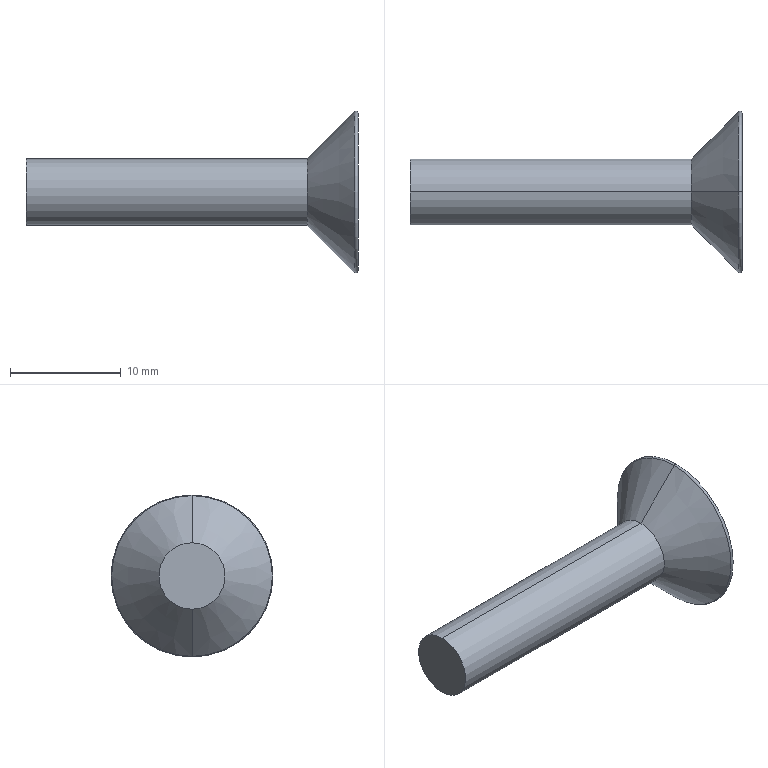Component | SolidWorks | FrontMiddleLowerDoor-1_hex lobular socket ctsk screws gb-2 | 1 solid | 20 faces | box 30 x 14.63 x 14.63 mm | volume 1112 mm3 | plane 14 | torus 2 | cone 2 | cylinder 2 | commonest cylinder face diameters 6 x2
STEP:
#1=COLOUR_RGB('',0.7922,0.8196,0.9333);
#2=FILL_AREA_STYLE_COLOUR('',#1);
#3=FILL_AREA_STYLE('',(#2));
#4=SURFACE_STYLE_FILL_AREA(#3);
#5=SURFACE_SIDE_STYLE('',(#4));
#6=SURFACE_STYLE_USAGE(.BOTH.,#5);
#7=PRESENTATION_STYLE_ASSIGNMENT((#6));
#8=CARTESIAN_POINT('',(16.378,12.559,-9.552));
#9=VERTEX_POINT('',#8);
#10=CARTESIAN_POINT('',(16.378,12.559,-8.991));
#11=VERTEX_POINT('',#10);
#12=CARTESIAN_POINT('',(16.378,12.559,-9.272));
#13=DIRECTION('',(1.,0.,-0.));
#14=DIRECTION('',(0.,0.,1.));
#15=AXIS2_PLACEMENT_3D('',#12,#13,#14);
#16=CIRCLE('',#15,0.2802);
#17=EDGE_CURVE('',#9,#11,#16,.T.);
#18=ORIENTED_EDGE('',*,*,#17,.F.);
#19=CARTESIAN_POINT('',(16.365,12.559,-9.557));
#20=VERTEX_POINT('',#19);
#21=CARTESIAN_POINT('',(16.37,12.559,-9.552));
#22=DIRECTION('',(-0.,1.,-0.));
#23=DIRECTION('',(-1.,0.,0.));
#24=AXIS2_PLACEMENT_3D('',#21,#22,#23);
#25=CIRCLE('',#24,0.007874);
#26=EDGE_CURVE('',#9,#20,#25,.T.);
#27=ORIENTED_EDGE('',*,*,#26,.T.);
#28=CARTESIAN_POINT('',(16.365,12.559,-8.986));
#29=VERTEX_POINT('',#28);
#30=CARTESIAN_POINT('',(16.365,12.559,-9.272));
#31=DIRECTION('',(-1.,-0.,0.));
#32=DIRECTION('',(0.,0.,-1.));
#33=AXIS2_PLACEMENT_3D('',#30,#31,#32);
#34=CIRCLE('',#33,0.2858);
#35=EDGE_CURVE('',#29,#20,#34,.T.);
#36=ORIENTED_EDGE('',*,*,#35,.F.);
#37=CARTESIAN_POINT('',(16.37,12.559,-8.991));
#38=DIRECTION('',(0.,-1.,0.));
#39=DIRECTION('',(0.,0.,-1.));
#40=AXIS2_PLACEMENT_3D('',#37,#38,#39);
#41=CIRCLE('',#40,0.007874);
#42=EDGE_CURVE('',#11,#29,#41,.T.);
#43=ORIENTED_EDGE('',*,*,#42,.F.);
#44=EDGE_LOOP('',(#18,#27,#36,#43));
#45=FACE_OUTER_BOUND('',#44,.T.);
#46=CARTESIAN_POINT('',(16.37,12.559,-9.272));
#47=DIRECTION('',(-1.,-0.,0.));
#48=DIRECTION('',(0.,0.,1.));
#49=AXIS2_PLACEMENT_3D('',#46,#47,#48);
#50=TOROIDAL_SURFACE('',#49,0.2802,0.007874);
#51=ADVANCED_FACE('',(#45),#50,.T.);
#52=CARTESIAN_POINT('',(16.197,12.559,-9.39));
#53=VERTEX_POINT('',#52);
#54=CARTESIAN_POINT('',(16.197,12.559,-9.154));
#55=VERTEX_POINT('',#54);
#56=CARTESIAN_POINT('',(16.197,12.559,-9.272));
#57=DIRECTION('',(-1.,-0.,0.));
#58=DIRECTION('',(0.,0.,1.));
#59=AXIS2_PLACEMENT_3D('',#56,#57,#58);
#60=CIRCLE('',#59,0.1181);
#61=EDGE_CURVE('',#53,#55,#60,.T.);
#62=ORIENTED_EDGE('',*,*,#61,.F.);
#63=CARTESIAN_POINT('',(16.197,12.559,-9.39));
#64=DIRECTION('',(0.7071,-0.,-0.7071));
#65=VECTOR('',#64,39.37);
#66=LINE('',#63,#65);
#67=EDGE_CURVE('',#53,#20,#66,.T.);
#68=ORIENTED_EDGE('',*,*,#67,.T.);
#69=CARTESIAN_POINT('',(16.365,12.559,-9.272));
#70=DIRECTION('',(-1.,-0.,0.));
#71=DIRECTION('',(0.,0.,-1.));
#72=AXIS2_PLACEMENT_3D('',#69,#70,#71);
#73=CIRCLE('',#72,0.2858);
#74=EDGE_CURVE('',#20,#29,#73,.T.);
#75=ORIENTED_EDGE('',*,*,#74,.T.);
#76=CARTESIAN_POINT('',(16.197,12.559,-9.154));
#77=DIRECTION('',(0.7071,0.,0.7071));
#78=VECTOR('',#77,39.37);
#79=LINE('',#76,#78);
#80=EDGE_CURVE('',#55,#29,#79,.T.);
#81=ORIENTED_EDGE('',*,*,#80,.F.);
#82=EDGE_LOOP('',(#62,#68,#75,#81));
#83=FACE_OUTER_BOUND('',#82,.T.);
#84=CARTESIAN_POINT('',(16.197,12.559,-9.272));
#85=DIRECTION('',(1.,0.,-0.));
#86=DIRECTION('',(0.,0.,1.));
#87=AXIS2_PLACEMENT_3D('',#84,#85,#86);
#88=CONICAL_SURFACE('',#87,0.1181,0.7854);
#89=ADVANCED_FACE('',(#83),#88,.T.);
#90=CARTESIAN_POINT('',(15.197,12.559,-9.154));
#91=VERTEX_POINT('',#90);
#92=CARTESIAN_POINT('',(15.197,12.559,-9.39));
#93=VERTEX_POINT('',#92);
#94=CARTESIAN_POINT('',(15.197,12.559,-9.272));
#95=DIRECTION('',(-1.,-0.,0.));
#96=DIRECTION('',(0.,0.,1.));
#97=AXIS2_PLACEMENT_3D('',#94,#95,#96);
#98=CIRCLE('',#97,0.1181);
#99=EDGE_CURVE('',#91,#93,#98,.T.);
#100=ORIENTED_EDGE('',*,*,#99,.F.);
#101=CARTESIAN_POINT('',(15.016,12.559,-9.154));
#102=DIRECTION('',(1.,0.,-0.));
#103=VECTOR('',#102,39.37);
#104=LINE('',#101,#103);
#105=EDGE_CURVE('',#91,#55,#104,.T.);
#106=ORIENTED_EDGE('',*,*,#105,.T.);
#107=CARTESIAN_POINT('',(16.197,12.559,-9.272));
#108=DIRECTION('',(-1.,-0.,0.));
#109=DIRECTION('',(0.,0.,1.));
#110=AXIS2_PLACEMENT_3D('',#107,#108,#109);
#111=CIRCLE('',#110,0.1181);
#112=EDGE_CURVE('',#55,#53,#111,.T.);
#113=ORIENTED_EDGE('',*,*,#112,.T.);
#114=CARTESIAN_POINT('',(15.016,12.559,-9.39));
#115=DIRECTION('',(1.,0.,-0.));
#116=VECTOR('',#115,39.37);
#117=LINE('',#114,#116);
#118=EDGE_CURVE('',#93,#53,#117,.T.);
#119=ORIENTED_EDGE('',*,*,#118,.F.);
#120=EDGE_LOOP('',(#100,#106,#113,#119));
#121=FACE_OUTER_BOUND('',#120,.T.);
#122=CARTESIAN_POINT('',(15.016,12.559,-9.272));
#123=DIRECTION('',(1.,0.,-0.));
#124=DIRECTION('',(0.,0.,-1.));
#125=AXIS2_PLACEMENT_3D('',#122,#123,#124);
#126=CYLINDRICAL_SURFACE('',#125,0.1181);
#127=ADVANCED_FACE('',(#121),#126,.T.);
#128=CARTESIAN_POINT('',(16.378,12.559,-9.272));
#129=DIRECTION('',(1.,0.,-0.));
#130=DIRECTION('',(0.,0.,1.));
#131=AXIS2_PLACEMENT_3D('',#128,#129,#130);
#132=CIRCLE('',#131,0.2802);
#133=EDGE_CURVE('',#11,#9,#132,.T.);
#134=ORIENTED_EDGE('',*,*,#133,.T.);
#135=ORIENTED_EDGE('',*,*,#17,.T.);
#136=EDGE_LOOP('',(#134,#135));
#137=FACE_OUTER_BOUND('',#136,.T.);
#138=CARTESIAN_POINT('',(16.378,12.477,-9.224));
#139=VERTEX_POINT('',#138);
#140=CARTESIAN_POINT('',(16.378,12.559,-9.177));
#141=VERTEX_POINT('',#140);
#142=CARTESIAN_POINT('',(16.378,12.477,-9.224));
#143=DIRECTION('',(0.,0.866,0.5));
#144=VECTOR('',#143,39.37);
#145=LINE('',#142,#144);
#146=EDGE_CURVE('',#139,#141,#145,.T.);
#147=ORIENTED_EDGE('',*,*,#146,.T.);
#148=CARTESIAN_POINT('',(16.378,12.641,-9.224));
#149=VERTEX_POINT('',#148);
#150=CARTESIAN_POINT('',(16.378,12.559,-9.177));
#151=DIRECTION('',(-0.,0.866,-0.5));
#152=VECTOR('',#151,39.37);
#153=LINE('',#150,#152);
#154=EDGE_CURVE('',#141,#149,#153,.T.);
#155=ORIENTED_EDGE('',*,*,#154,.T.);
#156=CARTESIAN_POINT('',(16.378,12.641,-9.319));
#157=VERTEX_POINT('',#156);
#158=CARTESIAN_POINT('',(16.378,12.641,-9.224));
#159=DIRECTION('',(-0.,-0.,-1.));
#160=VECTOR('',#159,39.37);
#161=LINE('',#158,#160);
#162=EDGE_CURVE('',#149,#157,#161,.T.);
#163=ORIENTED_EDGE('',*,*,#162,.T.);
#164=CARTESIAN_POINT('',(16.378,12.559,-9.366));
#165=VERTEX_POINT('',#164);
#166=CARTESIAN_POINT('',(16.378,12.641,-9.319));
#167=DIRECTION('',(-0.,-0.866,-0.5));
#168=VECTOR('',#167,39.37);
#169=LINE('',#166,#168);
#170=EDGE_CURVE('',#157,#165,#169,.T.);
#171=ORIENTED_EDGE('',*,*,#170,.T.);
#172=CARTESIAN_POINT('',(16.378,12.477,-9.319));
#173=VERTEX_POINT('',#172);
#174=CARTESIAN_POINT('',(16.378,12.559,-9.366));
#175=DIRECTION('',(0.,-0.866,0.5));
#176=VECTOR('',#175,39.37);
#177=LINE('',#174,#176);
#178=EDGE_CURVE('',#165,#173,#177,.T.);
#179=ORIENTED_EDGE('',*,*,#178,.T.);
#180=CARTESIAN_POINT('',(16.378,12.477,-9.319));
#181=DIRECTION('',(0.,0.,1.));
#182=VECTOR('',#181,39.37);
#183=LINE('',#180,#182);
#184=EDGE_CURVE('',#173,#139,#183,.T.);
#185=ORIENTED_EDGE('',*,*,#184,.T.);
#186=EDGE_LOOP('',(#147,#155,#163,#171,#179,#185));
#187=FACE_BOUND('',#186,.T.);
#188=CARTESIAN_POINT('',(16.378,12.559,-9.272));
#189=DIRECTION('',(-1.,-0.,0.));
#190=DIRECTION('',(0.,0.,1.));
#191=AXIS2_PLACEMENT_3D('',#188,#189,#190);
#192=PLANE('',#191);
#193=ADVANCED_FACE('',(#137,#187),#192,.F.);
#194=ORIENTED_EDGE('',*,*,#105,.F.);
#195=CARTESIAN_POINT('',(15.197,12.559,-9.272));
#196=DIRECTION('',(-1.,-0.,0.));
#197=DIRECTION('',(0.,0.,1.));
#198=AXIS2_PLACEMENT_3D('',#195,#196,#197);
#199=CIRCLE('',#198,0.1181);
#200=EDGE_CURVE('',#93,#91,#199,.T.);
#201=ORIENTED_EDGE('',*,*,#200,.F.);
#202=ORIENTED_EDGE('',*,*,#118,.T.);
#203=ORIENTED_EDGE('',*,*,#61,.T.);
#204=EDGE_LOOP('',(#194,#201,#202,#203));
#205=FACE_OUTER_BOUND('',#204,.T.);
#206=CARTESIAN_POINT('',(15.016,12.559,-9.272));
#207=DIRECTION('',(1.,0.,-0.));
#208=DIRECTION('',(0.,0.,-1.));
#209=AXIS2_PLACEMENT_3D('',#206,#207,#208);
#210=CYLINDRICAL_SURFACE('',#209,0.1181);
#211=ADVANCED_FACE('',(#205),#210,.T.);
#212=ORIENTED_EDGE('',*,*,#67,.F.);
#213=ORIENTED_EDGE('',*,*,#112,.F.);
#214=ORIENTED_EDGE('',*,*,#80,.T.);
#215=ORIENTED_EDGE('',*,*,#35,.T.);
#216=EDGE_LOOP('',(#212,#213,#214,#215));
#217=FACE_OUTER_BOUND('',#216,.T.);
#218=CARTESIAN_POINT('',(16.197,12.559,-9.272));
#219=DIRECTION('',(1.,0.,-0.));
#220=DIRECTION('',(0.,0.,1.));
#221=AXIS2_PLACEMENT_3D('',#218,#219,#220);
#222=CONICAL_SURFACE('',#221,0.1181,0.7854);
#223=ADVANCED_FACE('',(#217),#222,.T.);
#224=ORIENTED_EDGE('',*,*,#200,.T.);
#225=ORIENTED_EDGE('',*,*,#99,.T.);
#226=EDGE_LOOP('',(#224,#225));
#227=FACE_OUTER_BOUND('',#226,.T.);
#228=CARTESIAN_POINT('',(15.197,12.795,-11.65));
#229=DIRECTION('',(-1.,-0.,0.));
#230=DIRECTION('',(0.,0.,1.));
#231=AXIS2_PLACEMENT_3D('',#228,#229,#230);
#232=PLANE('',#231);
#233=ADVANCED_FACE('',(#227),#232,.T.);
#234=ORIENTED_EDGE('',*,*,#146,.F.);
#235=CARTESIAN_POINT('',(16.299,12.477,-9.224));
#236=VERTEX_POINT('',#235);
#237=CARTESIAN_POINT('',(16.299,12.477,-9.224));
#238=DIRECTION('',(1.,0.,-0.));
#239=VECTOR('',#238,39.37);
#240=LINE('',#237,#239);
#241=EDGE_CURVE('',#236,#139,#240,.T.);
#242=ORIENTED_EDGE('',*,*,#241,.F.);
#243=CARTESIAN_POINT('',(16.299,12.559,-9.177));
#244=VERTEX_POINT('',#243);
#245=CARTESIAN_POINT('',(16.299,12.477,-9.224));
#246=DIRECTION('',(0.,0.866,0.5));
#247=VECTOR('',#246,39.37);
#248=LINE('',#245,#247);
#249=EDGE_CURVE('',#236,#244,#248,.T.);
#250=ORIENTED_EDGE('',*,*,#249,.T.);
#251=CARTESIAN_POINT('',(16.299,12.559,-9.177));
#252=DIRECTION('',(1.,0.,-0.));
#253=VECTOR('',#252,39.37);
#254=LINE('',#251,#253);
#255=EDGE_CURVE('',#244,#141,#254,.T.);
#256=ORIENTED_EDGE('',*,*,#255,.T.);
#257=EDGE_LOOP('',(#234,#242,#250,#256));
#258=FACE_OUTER_BOUND('',#257,.T.);
#259=CARTESIAN_POINT('',(16.299,12.477,-9.224));
#260=DIRECTION('',(-0.,0.5,-0.866));
#261=DIRECTION('',(-0.,-0.866,-0.5));
#262=AXIS2_PLACEMENT_3D('',#259,#260,#261);
#263=PLANE('',#262);
#264=ADVANCED_FACE('',(#258),#263,.T.);
#265=ORIENTED_EDGE('',*,*,#154,.F.);
#266=ORIENTED_EDGE('',*,*,#255,.F.);
#267=CARTESIAN_POINT('',(16.299,12.641,-9.224));
#268=VERTEX_POINT('',#267);
#269=CARTESIAN_POINT('',(16.299,12.559,-9.177));
#270=DIRECTION('',(-0.,0.866,-0.5));
#271=VECTOR('',#270,39.37);
#272=LINE('',#269,#271);
#273=EDGE_CURVE('',#244,#268,#272,.T.);
#274=ORIENTED_EDGE('',*,*,#273,.T.);
#275=CARTESIAN_POINT('',(16.299,12.641,-9.224));
#276=DIRECTION('',(1.,0.,-0.));
#277=VECTOR('',#276,39.37);
#278=LINE('',#275,#277);
#279=EDGE_CURVE('',#268,#149,#278,.T.);
#280=ORIENTED_EDGE('',*,*,#279,.T.);
#281=EDGE_LOOP('',(#265,#266,#274,#280));
#282=FACE_OUTER_BOUND('',#281,.T.);
#283=CARTESIAN_POINT('',(16.299,12.559,-9.177));
#284=DIRECTION('',(-0.,-0.5,-0.866));
#285=DIRECTION('',(0.,-0.866,0.5));
#286=AXIS2_PLACEMENT_3D('',#283,#284,#285);
#287=PLANE('',#286);
#288=ADVANCED_FACE('',(#282),#287,.T.);
#289=ORIENTED_EDGE('',*,*,#162,.F.);
#290=ORIENTED_EDGE('',*,*,#279,.F.);
#291=CARTESIAN_POINT('',(16.299,12.641,-9.319));
#292=VERTEX_POINT('',#291);
#293=CARTESIAN_POINT('',(16.299,12.641,-9.224));
#294=DIRECTION('',(-0.,-0.,-1.));
#295=VECTOR('',#294,39.37);
#296=LINE('',#293,#295);
#297=EDGE_CURVE('',#268,#292,#296,.T.);
#298=ORIENTED_EDGE('',*,*,#297,.T.);
#299=CARTESIAN_POINT('',(16.299,12.641,-9.319));
#300=DIRECTION('',(1.,0.,-0.));
#301=VECTOR('',#300,39.37);
#302=LINE('',#299,#301);
#303=EDGE_CURVE('',#292,#157,#302,.T.);
#304=ORIENTED_EDGE('',*,*,#303,.T.);
#305=EDGE_LOOP('',(#289,#290,#298,#304));
#306=FACE_OUTER_BOUND('',#305,.T.);
#307=CARTESIAN_POINT('',(16.299,12.641,-9.224));
#308=DIRECTION('',(0.,-1.,0.));
#309=DIRECTION('',(0.,0.,1.));
#310=AXIS2_PLACEMENT_3D('',#307,#308,#309);
#311=PLANE('',#310);
#312=ADVANCED_FACE('',(#306),#311,.T.);
#313=ORIENTED_EDGE('',*,*,#170,.F.);
#314=ORIENTED_EDGE('',*,*,#303,.F.);
#315=CARTESIAN_POINT('',(16.299,12.559,-9.366));
#316=VERTEX_POINT('',#315);
#317=CARTESIAN_POINT('',(16.299,12.641,-9.319));
#318=DIRECTION('',(-0.,-0.866,-0.5));
#319=VECTOR('',#318,39.37);
#320=LINE('',#317,#319);
#321=EDGE_CURVE('',#292,#316,#320,.T.);
#322=ORIENTED_EDGE('',*,*,#321,.T.);
#323=CARTESIAN_POINT('',(16.299,12.559,-9.366));
#324=DIRECTION('',(1.,0.,-0.));
#325=VECTOR('',#324,39.37);
#326=LINE('',#323,#325);
#327=EDGE_CURVE('',#316,#165,#326,.T.);
#328=ORIENTED_EDGE('',*,*,#327,.T.);
#329=EDGE_LOOP('',(#313,#314,#322,#328));
#330=FACE_OUTER_BOUND('',#329,.T.);
#331=CARTESIAN_POINT('',(16.299,12.641,-9.319));
#332=DIRECTION('',(0.,-0.5,0.866));
#333=DIRECTION('',(0.,0.866,0.5));
#334=AXIS2_PLACEMENT_3D('',#331,#332,#333);
#335=PLANE('',#334);
#336=ADVANCED_FACE('',(#330),#335,.T.);
#337=ORIENTED_EDGE('',*,*,#178,.F.);
#338=ORIENTED_EDGE('',*,*,#327,.F.);
#339=CARTESIAN_POINT('',(16.299,12.477,-9.319));
#340=VERTEX_POINT('',#339);
#341=CARTESIAN_POINT('',(16.299,12.559,-9.366));
#342=DIRECTION('',(0.,-0.866,0.5));
#343=VECTOR('',#342,39.37);
#344=LINE('',#341,#343);
#345=EDGE_CURVE('',#316,#340,#344,.T.);
#346=ORIENTED_EDGE('',*,*,#345,.T.);
#347=CARTESIAN_POINT('',(16.299,12.477,-9.319));
#348=DIRECTION('',(1.,0.,-0.));
#349=VECTOR('',#348,39.37);
#350=LINE('',#347,#349);
#351=EDGE_CURVE('',#340,#173,#350,.T.);
#352=ORIENTED_EDGE('',*,*,#351,.T.);
#353=EDGE_LOOP('',(#337,#338,#346,#352));
#354=FACE_OUTER_BOUND('',#353,.T.);
#355=CARTESIAN_POINT('',(16.299,12.559,-9.366));
#356=DIRECTION('',(0.,0.5,0.866));
#357=DIRECTION('',(-0.,0.866,-0.5));
#358=AXIS2_PLACEMENT_3D('',#355,#356,#357);
#359=PLANE('',#358);
#360=ADVANCED_FACE('',(#354),#359,.T.);
#361=ORIENTED_EDGE('',*,*,#184,.F.);
#362=ORIENTED_EDGE('',*,*,#351,.F.);
#363=CARTESIAN_POINT('',(16.299,12.477,-9.319));
#364=DIRECTION('',(0.,0.,1.));
#365=VECTOR('',#364,39.37);
#366=LINE('',#363,#365);
#367=EDGE_CURVE('',#340,#236,#366,.T.);
#368=ORIENTED_EDGE('',*,*,#367,.T.);
#369=ORIENTED_EDGE('',*,*,#241,.T.);
#370=EDGE_LOOP('',(#361,#362,#368,#369));
#371=FACE_OUTER_BOUND('',#370,.T.);
#372=CARTESIAN_POINT('',(16.299,12.477,-9.319));
#373=DIRECTION('',(-0.,1.,-0.));
#374=DIRECTION('',(-0.,-0.,-1.));
#375=AXIS2_PLACEMENT_3D('',#372,#373,#374);
#376=PLANE('',#375);
#377=ADVANCED_FACE('',(#371),#376,.T.);
#378=ORIENTED_EDGE('',*,*,#273,.F.);
#379=CARTESIAN_POINT('',(16.252,12.559,-9.272));
#380=VERTEX_POINT('',#379);
#381=CARTESIAN_POINT('',(16.299,12.559,-9.177));
#382=DIRECTION('',(0.4472,0.,0.8944));
#383=VECTOR('',#382,39.37);
#384=LINE('',#381,#383);
#385=EDGE_CURVE('',#380,#244,#384,.T.);
#386=ORIENTED_EDGE('',*,*,#385,.F.);
#387=CARTESIAN_POINT('',(16.299,12.641,-9.224));
#388=DIRECTION('',(0.4472,0.7746,0.4472));
#389=VECTOR('',#388,39.37);
#390=LINE('',#387,#389);
#391=EDGE_CURVE('',#380,#268,#390,.T.);
#392=ORIENTED_EDGE('',*,*,#391,.T.);
#393=EDGE_LOOP('',(#378,#386,#392));
#394=FACE_OUTER_BOUND('',#393,.T.);
#395=CARTESIAN_POINT('',(16.299,12.559,-9.177));
#396=DIRECTION('',(-0.866,0.25,0.433));
#397=DIRECTION('',(0.4472,0.,0.8944));
#398=AXIS2_PLACEMENT_3D('',#395,#396,#397);
#399=PLANE('',#398);
#400=ADVANCED_FACE('',(#394),#399,.F.);
#401=ORIENTED_EDGE('',*,*,#297,.F.);
#402=ORIENTED_EDGE('',*,*,#391,.F.);
#403=CARTESIAN_POINT('',(16.299,12.641,-9.319));
#404=DIRECTION('',(0.4472,0.7746,-0.4472));
#405=VECTOR('',#404,39.37);
#406=LINE('',#403,#405);
#407=EDGE_CURVE('',#380,#292,#406,.T.);
#408=ORIENTED_EDGE('',*,*,#407,.T.);
#409=EDGE_LOOP('',(#401,#402,#408));
#410=FACE_OUTER_BOUND('',#409,.T.);
#411=CARTESIAN_POINT('',(16.299,12.641,-9.224));
#412=DIRECTION('',(-0.866,0.5,0.));
#413=DIRECTION('',(0.5,0.866,-0.));
#414=AXIS2_PLACEMENT_3D('',#411,#412,#413);
#415=PLANE('',#414);
#416=ADVANCED_FACE('',(#410),#415,.F.);
#417=ORIENTED_EDGE('',*,*,#321,.F.);
#418=ORIENTED_EDGE('',*,*,#407,.F.);
#419=CARTESIAN_POINT('',(16.299,12.559,-9.366));
#420=DIRECTION('',(0.4472,-0.,-0.8944));
#421=VECTOR('',#420,39.37);
#422=LINE('',#419,#421);
#423=EDGE_CURVE('',#380,#316,#422,.T.);
#424=ORIENTED_EDGE('',*,*,#423,.T.);
#425=EDGE_LOOP('',(#417,#418,#424));
#426=FACE_OUTER_BOUND('',#425,.T.);
#427=CARTESIAN_POINT('',(16.299,12.641,-9.319));
#428=DIRECTION('',(-0.866,0.25,-0.433));
#429=DIRECTION('',(-0.4472,0.,0.8944));
#430=AXIS2_PLACEMENT_3D('',#427,#428,#429);
#431=PLANE('',#430);
#432=ADVANCED_FACE('',(#426),#431,.F.);
#433=ORIENTED_EDGE('',*,*,#345,.F.);
#434=ORIENTED_EDGE('',*,*,#423,.F.);
#435=CARTESIAN_POINT('',(16.299,12.477,-9.319));
#436=DIRECTION('',(0.4472,-0.7746,-0.4472));
#437=VECTOR('',#436,39.37);
#438=LINE('',#435,#437);
#439=EDGE_CURVE('',#380,#340,#438,.T.);
#440=ORIENTED_EDGE('',*,*,#439,.T.);
#441=EDGE_LOOP('',(#433,#434,#440));
#442=FACE_OUTER_BOUND('',#441,.T.);
#443=CARTESIAN_POINT('',(16.299,12.559,-9.366));
#444=DIRECTION('',(-0.866,-0.25,-0.433));
#445=DIRECTION('',(-0.4472,0.,0.8944));
#446=AXIS2_PLACEMENT_3D('',#443,#444,#445);
#447=PLANE('',#446);
#448=ADVANCED_FACE('',(#442),#447,.F.);
#449=ORIENTED_EDGE('',*,*,#367,.F.);
#450=ORIENTED_EDGE('',*,*,#439,.F.);
#451=CARTESIAN_POINT('',(16.299,12.477,-9.224));
#452=DIRECTION('',(0.4472,-0.7746,0.4472));
#453=VECTOR('',#452,39.37);
#454=LINE('',#451,#453);
#455=EDGE_CURVE('',#380,#236,#454,.T.);
#456=ORIENTED_EDGE('',*,*,#455,.T.);
#457=EDGE_LOOP('',(#449,#450,#456));
#458=FACE_OUTER_BOUND('',#457,.T.);
#459=CARTESIAN_POINT('',(16.299,12.477,-9.319));
#460=DIRECTION('',(-0.866,-0.5,0.));
#461=DIRECTION('',(-0.5,0.866,0.));
#462=AXIS2_PLACEMENT_3D('',#459,#460,#461);
#463=PLANE('',#462);
#464=ADVANCED_FACE('',(#458),#463,.F.);
#465=ORIENTED_EDGE('',*,*,#249,.F.);
#466=ORIENTED_EDGE('',*,*,#455,.F.);
#467=ORIENTED_EDGE('',*,*,#385,.T.);
#468=EDGE_LOOP('',(#465,#466,#467));
#469=FACE_OUTER_BOUND('',#468,.T.);
#470=CARTESIAN_POINT('',(16.299,12.477,-9.224));
#471=DIRECTION('',(-0.866,-0.25,0.433));
#472=DIRECTION('',(0.4472,0.,0.8944));
#473=AXIS2_PLACEMENT_3D('',#470,#471,#472);
#474=PLANE('',#473);
#475=ADVANCED_FACE('',(#469),#474,.F.);
#476=ORIENTED_EDGE('',*,*,#26,.F.);
#477=ORIENTED_EDGE('',*,*,#133,.F.);
#478=ORIENTED_EDGE('',*,*,#42,.T.);
#479=ORIENTED_EDGE('',*,*,#74,.F.);
#480=EDGE_LOOP('',(#476,#477,#478,#479));
#481=FACE_OUTER_BOUND('',#480,.T.);
#482=CARTESIAN_POINT('',(16.37,12.559,-9.272));
#483=DIRECTION('',(-1.,-0.,0.));
#484=DIRECTION('',(0.,0.,1.));
#485=AXIS2_PLACEMENT_3D('',#482,#483,#484);
#486=TOROIDAL_SURFACE('',#485,0.2802,0.007874);
#487=ADVANCED_FACE('',(#481),#486,.T.);
#488=CLOSED_SHELL('',(#51,#89,#127,#193,#211,#223,#233,#264,#288,#312,#336,#360,#377,#400,#416,#432,#448,#464,#475,#487));
#489=MANIFOLD_SOLID_BREP('',#488);
#490=STYLED_ITEM('',(#7),#489);
#491=(LENGTH_UNIT()NAMED_UNIT(*)SI_UNIT($,.METRE.));
#492=LENGTH_MEASURE_WITH_UNIT(LENGTH_MEASURE(0.0254),#491);
#493=DIMENSIONAL_EXPONENTS(1.,0.,0.,0.,0.,0.,0.);
#494=(CONVERSION_BASED_UNIT('',#492)LENGTH_UNIT()NAMED_UNIT(#493));
#495=UNCERTAINTY_MEASURE_WITH_UNIT(LENGTH_MEASURE(0.00001),#494,'','');
#496=(NAMED_UNIT(*)PLANE_ANGLE_UNIT()SI_UNIT($,.RADIAN.));
#497=(NAMED_UNIT(*)SI_UNIT($,.STERADIAN.)SOLID_ANGLE_UNIT());
#498=(GEOMETRIC_REPRESENTATION_CONTEXT(3)GLOBAL_UNCERTAINTY_ASSIGNED_CONTEXT((#495))GLOBAL_UNIT_ASSIGNED_CONTEXT((#494,#496,#497))REPRESENTATION_CONTEXT('',''));
#499=MECHANICAL_DESIGN_GEOMETRIC_PRESENTATION_REPRESENTATION('',(#490),#498);
#500=PRESENTATION_LAYER_ASSIGNMENT('','',(#490));
#501=CARTESIAN_POINT('',(0.,0.,0.));
#502=DIRECTION('',(0.,0.,1.));
#503=DIRECTION('',(1.,0.,0.));
#504=AXIS2_PLACEMENT_3D('',#501,#502,#503);
#505=(LENGTH_UNIT()NAMED_UNIT(*)SI_UNIT($,.METRE.));
#506=LENGTH_MEASURE_WITH_UNIT(LENGTH_MEASURE(0.0254),#505);
#507=DIMENSIONAL_EXPONENTS(1.,0.,0.,0.,0.,0.,0.);
#508=(CONVERSION_BASED_UNIT('',#506)LENGTH_UNIT()NAMED_UNIT(#507));
#509=UNCERTAINTY_MEASURE_WITH_UNIT(LENGTH_MEASURE(0.00001),#508,'','');
#510=(NAMED_UNIT(*)PLANE_ANGLE_UNIT()SI_UNIT($,.RADIAN.));
#511=(NAMED_UNIT(*)SI_UNIT($,.STERADIAN.)SOLID_ANGLE_UNIT());
#512=(GEOMETRIC_REPRESENTATION_CONTEXT(3)GLOBAL_UNCERTAINTY_ASSIGNED_CONTEXT((#509))GLOBAL_UNIT_ASSIGNED_CONTEXT((#508,#510,#511))REPRESENTATION_CONTEXT('',''));
#513=ADVANCED_BREP_SHAPE_REPRESENTATION('',(#489,#504),#512);